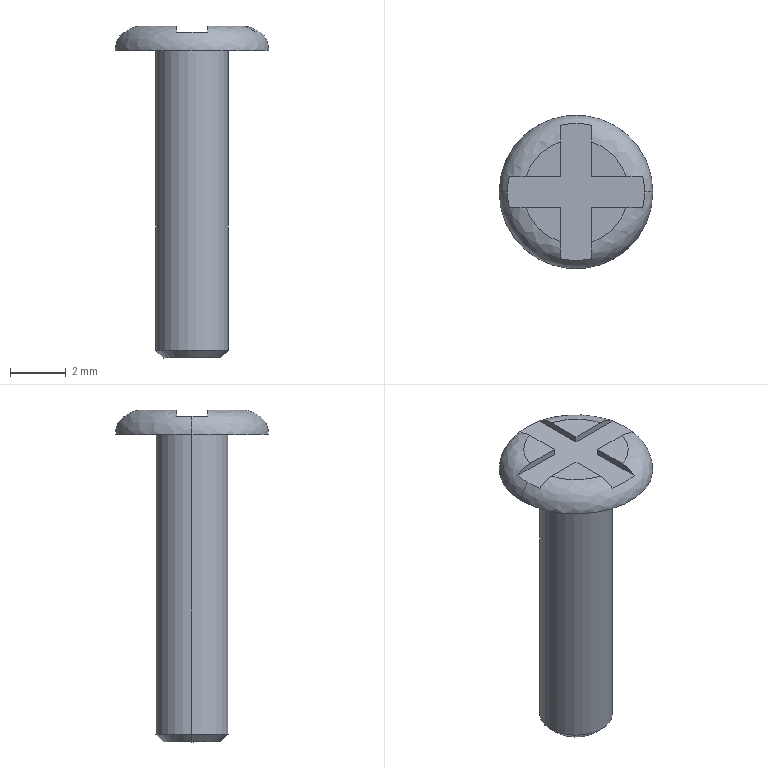Component | SolidWorks | NewCurveBenderHG20Slider-DoubleWheel-1_NewTypeCurveBenderHG20-DoubleWheel-1 | 1 solid | 21 faces | box 5.5 x 5.5 x 11.88 mm | volume 74 mm3 | plane 15 | spline 2 | cylinder 2 | cone 2 | commonest cylinder face diameters 2.6 x2
STEP:
#1=COLOUR_RGB('',0.7922,0.8196,0.9333);
#2=FILL_AREA_STYLE_COLOUR('',#1);
#3=FILL_AREA_STYLE('',(#2));
#4=SURFACE_STYLE_FILL_AREA(#3);
#5=SURFACE_SIDE_STYLE('',(#4));
#6=SURFACE_STYLE_USAGE(.BOTH.,#5);
#7=PRESENTATION_STYLE_ASSIGNMENT((#6));
#8=CARTESIAN_POINT('',(2.62,1.938,5.006));
#9=VERTEX_POINT('',#8);
#10=CARTESIAN_POINT('',(2.404,1.938,5.006));
#11=VERTEX_POINT('',#10);
#12=CARTESIAN_POINT('',(2.512,1.938,5.006));
#13=DIRECTION('',(-0.,0.,1.));
#14=DIRECTION('',(1.,0.,0.));
#15=AXIS2_PLACEMENT_3D('',#12,#13,#14);
#16=CIRCLE('',#15,0.1083);
#17=EDGE_CURVE('',#9,#11,#16,.T.);
#18=ORIENTED_EDGE('',*,*,#17,.T.);
#19=CARTESIAN_POINT('',(2.415,1.938,5.031));
#20=VERTEX_POINT('',#19);
#21=CARTESIAN_POINT('',(2.438,1.938,5.006));
#22=DIRECTION('',(-0.,1.,-0.));
#23=DIRECTION('',(-1.,0.,0.));
#24=AXIS2_PLACEMENT_3D('',#21,#22,#23);
#25=CIRCLE('',#24,0.03465);
#26=EDGE_CURVE('',#11,#20,#25,.T.);
#27=ORIENTED_EDGE('',*,*,#26,.T.);
#28=CARTESIAN_POINT('',(2.418,1.959,5.031));
#29=VERTEX_POINT('',#28);
#30=CARTESIAN_POINT('',(2.512,1.938,5.031));
#31=DIRECTION('',(0.,0.,-1.));
#32=DIRECTION('',(1.,0.,0.));
#33=AXIS2_PLACEMENT_3D('',#30,#31,#32);
#34=CIRCLE('',#33,0.09654);
#35=EDGE_CURVE('',#20,#29,#34,.T.);
#36=ORIENTED_EDGE('',*,*,#35,.T.);
#37=CARTESIAN_POINT('',(2.442,1.959,5.04));
#38=VERTEX_POINT('',#37);
#39=CARTESIAN_POINT('',(2.442,1.959,5.04));
#40=CARTESIAN_POINT('',(2.433,1.959,5.04));
#41=CARTESIAN_POINT('',(2.424,1.959,5.037));
#42=CARTESIAN_POINT('',(2.418,1.959,5.031));
#43=B_SPLINE_CURVE_WITH_KNOTS('',3,(#39,#40,#41,#42),.UNSPECIFIED.,.F.,.F.,(4,4),(0.,0.0006526),.UNSPECIFIED.);
#44=EDGE_CURVE('',#38,#29,#43,.T.);
#45=ORIENTED_EDGE('',*,*,#44,.F.);
#46=CARTESIAN_POINT('',(2.49,2.008,5.04));
#47=VERTEX_POINT('',#46);
#48=CARTESIAN_POINT('',(2.442,1.959,5.04));
#49=CARTESIAN_POINT('',(2.449,1.983,5.04));
#50=CARTESIAN_POINT('',(2.467,2.001,5.04));
#51=CARTESIAN_POINT('',(2.49,2.008,5.04));
#52=(BOUNDED_CURVE()B_SPLINE_CURVE(3,(#48,#49,#50,#51),.UNSPECIFIED.,.F.,.F.)B_SPLINE_CURVE_WITH_KNOTS((4,4),(0.,1.),.UNSPECIFIED.)CURVE()GEOMETRIC_REPRESENTATION_ITEM()RATIONAL_B_SPLINE_CURVE((1.,0.9225,0.9225,1.))REPRESENTATION_ITEM(''));
#53=EDGE_CURVE('',#38,#47,#52,.T.);
#54=ORIENTED_EDGE('',*,*,#53,.T.);
#55=CARTESIAN_POINT('',(2.49,2.032,5.031));
#56=VERTEX_POINT('',#55);
#57=CARTESIAN_POINT('',(2.49,2.032,5.031));
#58=CARTESIAN_POINT('',(2.49,2.025,5.037));
#59=CARTESIAN_POINT('',(2.49,2.017,5.04));
#60=CARTESIAN_POINT('',(2.49,2.008,5.04));
#61=B_SPLINE_CURVE_WITH_KNOTS('',3,(#57,#58,#59,#60),.UNSPECIFIED.,.F.,.F.,(4,4),(0.,0.0006513),.UNSPECIFIED.);
#62=EDGE_CURVE('',#56,#47,#61,.T.);
#63=ORIENTED_EDGE('',*,*,#62,.F.);
#64=CARTESIAN_POINT('',(2.534,2.032,5.031));
#65=VERTEX_POINT('',#64);
#66=CARTESIAN_POINT('',(2.512,1.938,5.031));
#67=DIRECTION('',(0.,0.,-1.));
#68=DIRECTION('',(1.,0.,0.));
#69=AXIS2_PLACEMENT_3D('',#66,#67,#68);
#70=CIRCLE('',#69,0.09654);
#71=EDGE_CURVE('',#56,#65,#70,.T.);
#72=ORIENTED_EDGE('',*,*,#71,.T.);
#73=CARTESIAN_POINT('',(2.534,2.008,5.04));
#74=VERTEX_POINT('',#73);
#75=CARTESIAN_POINT('',(2.534,2.008,5.04));
#76=CARTESIAN_POINT('',(2.534,2.017,5.04));
#77=CARTESIAN_POINT('',(2.534,2.025,5.037));
#78=CARTESIAN_POINT('',(2.534,2.032,5.031));
#79=B_SPLINE_CURVE_WITH_KNOTS('',3,(#75,#76,#77,#78),.UNSPECIFIED.,.F.,.F.,(4,4),(0.,0.0006526),.UNSPECIFIED.);
#80=EDGE_CURVE('',#74,#65,#79,.T.);
#81=ORIENTED_EDGE('',*,*,#80,.F.);
#82=CARTESIAN_POINT('',(2.582,1.959,5.04));
#83=VERTEX_POINT('',#82);
#84=CARTESIAN_POINT('',(2.534,2.008,5.04));
#85=CARTESIAN_POINT('',(2.557,2.001,5.04));
#86=CARTESIAN_POINT('',(2.575,1.983,5.04));
#87=CARTESIAN_POINT('',(2.582,1.959,5.04));
#88=(BOUNDED_CURVE()B_SPLINE_CURVE(3,(#84,#85,#86,#87),.UNSPECIFIED.,.F.,.F.)B_SPLINE_CURVE_WITH_KNOTS((4,4),(0.,1.),.UNSPECIFIED.)CURVE()GEOMETRIC_REPRESENTATION_ITEM()RATIONAL_B_SPLINE_CURVE((1.,0.9225,0.9225,1.))REPRESENTATION_ITEM(''));
#89=EDGE_CURVE('',#74,#83,#88,.T.);
#90=ORIENTED_EDGE('',*,*,#89,.T.);
#91=CARTESIAN_POINT('',(2.606,1.959,5.031));
#92=VERTEX_POINT('',#91);
#93=CARTESIAN_POINT('',(2.606,1.959,5.031));
#94=CARTESIAN_POINT('',(2.599,1.959,5.037));
#95=CARTESIAN_POINT('',(2.591,1.959,5.04));
#96=CARTESIAN_POINT('',(2.582,1.959,5.04));
#97=B_SPLINE_CURVE_WITH_KNOTS('',3,(#93,#94,#95,#96),.UNSPECIFIED.,.F.,.F.,(4,4),(0.,0.0006513),.UNSPECIFIED.);
#98=EDGE_CURVE('',#92,#83,#97,.T.);
#99=ORIENTED_EDGE('',*,*,#98,.F.);
#100=CARTESIAN_POINT('',(2.609,1.938,5.031));
#101=VERTEX_POINT('',#100);
#102=CARTESIAN_POINT('',(2.512,1.938,5.031));
#103=DIRECTION('',(0.,0.,-1.));
#104=DIRECTION('',(1.,0.,0.));
#105=AXIS2_PLACEMENT_3D('',#102,#103,#104);
#106=CIRCLE('',#105,0.09654);
#107=EDGE_CURVE('',#92,#101,#106,.T.);
#108=ORIENTED_EDGE('',*,*,#107,.T.);
#109=CARTESIAN_POINT('',(2.586,1.938,5.006));
#110=DIRECTION('',(0.,-1.,0.));
#111=DIRECTION('',(1.,0.,0.));
#112=AXIS2_PLACEMENT_3D('',#109,#110,#111);
#113=CIRCLE('',#112,0.03465);
#114=EDGE_CURVE('',#9,#101,#113,.T.);
#115=ORIENTED_EDGE('',*,*,#114,.F.);
#116=EDGE_LOOP('',(#18,#27,#36,#45,#54,#63,#72,#81,#90,#99,#108,#115));
#117=FACE_OUTER_BOUND('',#116,.T.);
#118=CARTESIAN_POINT('',(2.404,1.938,5.006));
#119=CARTESIAN_POINT('',(2.404,2.154,5.006));
#120=CARTESIAN_POINT('',(2.62,2.154,5.006));
#121=CARTESIAN_POINT('',(2.62,1.938,5.006));
#122=CARTESIAN_POINT('',(2.404,1.938,5.026));
#123=CARTESIAN_POINT('',(2.404,2.154,5.026));
#124=CARTESIAN_POINT('',(2.62,2.154,5.026));
#125=CARTESIAN_POINT('',(2.62,1.938,5.026));
#126=CARTESIAN_POINT('',(2.418,1.938,5.04));
#127=CARTESIAN_POINT('',(2.418,2.125,5.04));
#128=CARTESIAN_POINT('',(2.606,2.125,5.04));
#129=CARTESIAN_POINT('',(2.606,1.938,5.04));
#130=CARTESIAN_POINT('',(2.438,1.938,5.04));
#131=CARTESIAN_POINT('',(2.438,2.085,5.04));
#132=CARTESIAN_POINT('',(2.586,2.085,5.04));
#133=CARTESIAN_POINT('',(2.586,1.938,5.04));
#134=(BOUNDED_SURFACE()B_SPLINE_SURFACE(3,3,((#118,#119,#120,#121),(#122,#123,#124,#125),(#126,#127,#128,#129),(#130,#131,#132,#133)),.UNSPECIFIED.,.F.,.F.,.F.)B_SPLINE_SURFACE_WITH_KNOTS((4,4),(4,4),(0.,1.),(0.,1.),.UNSPECIFIED.)GEOMETRIC_REPRESENTATION_ITEM()RATIONAL_B_SPLINE_SURFACE(((1.,0.3333,0.3333,1.),(0.8047,0.2682,0.2682,0.8047),(0.8047,0.2682,0.2682,0.8047),(1.,0.3333,0.3333,1.)))REPRESENTATION_ITEM('')SURFACE());
#135=ADVANCED_FACE('',(#117),#134,.T.);
#136=CARTESIAN_POINT('',(2.461,1.938,4.583));
#137=VERTEX_POINT('',#136);
#138=CARTESIAN_POINT('',(2.563,1.938,4.583));
#139=VERTEX_POINT('',#138);
#140=CARTESIAN_POINT('',(2.512,1.938,4.583));
#141=DIRECTION('',(-0.,0.,1.));
#142=DIRECTION('',(-1.,0.,-0.));
#143=AXIS2_PLACEMENT_3D('',#140,#141,#142);
#144=CIRCLE('',#143,0.05118);
#145=EDGE_CURVE('',#137,#139,#144,.T.);
#146=ORIENTED_EDGE('',*,*,#145,.T.);
#147=CARTESIAN_POINT('',(2.563,1.938,5.006));
#148=VERTEX_POINT('',#147);
#149=CARTESIAN_POINT('',(2.563,1.938,4.572));
#150=DIRECTION('',(-0.,0.,1.));
#151=VECTOR('',#150,39.37);
#152=LINE('',#149,#151);
#153=EDGE_CURVE('',#139,#148,#152,.T.);
#154=ORIENTED_EDGE('',*,*,#153,.T.);
#155=CARTESIAN_POINT('',(2.461,1.938,5.006));
#156=VERTEX_POINT('',#155);
#157=CARTESIAN_POINT('',(2.512,1.938,5.006));
#158=DIRECTION('',(0.,0.,-1.));
#159=DIRECTION('',(-1.,0.,0.));
#160=AXIS2_PLACEMENT_3D('',#157,#158,#159);
#161=CIRCLE('',#160,0.05118);
#162=EDGE_CURVE('',#148,#156,#161,.T.);
#163=ORIENTED_EDGE('',*,*,#162,.T.);
#164=CARTESIAN_POINT('',(2.461,1.938,4.572));
#165=DIRECTION('',(-0.,0.,1.));
#166=VECTOR('',#165,39.37);
#167=LINE('',#164,#166);
#168=EDGE_CURVE('',#137,#156,#167,.T.);
#169=ORIENTED_EDGE('',*,*,#168,.F.);
#170=EDGE_LOOP('',(#146,#154,#163,#169));
#171=FACE_OUTER_BOUND('',#170,.T.);
#172=CARTESIAN_POINT('',(2.512,1.938,4.572));
#173=DIRECTION('',(-0.,0.,1.));
#174=DIRECTION('',(-1.,0.,-0.));
#175=AXIS2_PLACEMENT_3D('',#172,#173,#174);
#176=CYLINDRICAL_SURFACE('',#175,0.05118);
#177=ADVANCED_FACE('',(#171),#176,.T.);
#178=CARTESIAN_POINT('',(2.472,1.938,4.572));
#179=VERTEX_POINT('',#178);
#180=CARTESIAN_POINT('',(2.552,1.938,4.572));
#181=VERTEX_POINT('',#180);
#182=CARTESIAN_POINT('',(2.512,1.938,4.572));
#183=DIRECTION('',(-0.,0.,1.));
#184=DIRECTION('',(-1.,0.,-0.));
#185=AXIS2_PLACEMENT_3D('',#182,#183,#184);
#186=CIRCLE('',#185,0.04031);
#187=EDGE_CURVE('',#179,#181,#186,.T.);
#188=ORIENTED_EDGE('',*,*,#187,.T.);
#189=CARTESIAN_POINT('',(2.563,1.938,4.583));
#190=DIRECTION('',(0.7071,-0.,0.7071));
#191=VECTOR('',#190,39.37);
#192=LINE('',#189,#191);
#193=EDGE_CURVE('',#181,#139,#192,.T.);
#194=ORIENTED_EDGE('',*,*,#193,.T.);
#195=ORIENTED_EDGE('',*,*,#145,.F.);
#196=CARTESIAN_POINT('',(2.461,1.938,4.583));
#197=DIRECTION('',(-0.7071,0.,0.7071));
#198=VECTOR('',#197,39.37);
#199=LINE('',#196,#198);
#200=EDGE_CURVE('',#179,#137,#199,.T.);
#201=ORIENTED_EDGE('',*,*,#200,.F.);
#202=EDGE_LOOP('',(#188,#194,#195,#201));
#203=FACE_OUTER_BOUND('',#202,.T.);
#204=CARTESIAN_POINT('',(2.512,1.938,4.583));
#205=DIRECTION('',(-0.,0.,1.));
#206=DIRECTION('',(-1.,0.,-0.));
#207=AXIS2_PLACEMENT_3D('',#204,#205,#206);
#208=CONICAL_SURFACE('',#207,0.05118,0.7854);
#209=ADVANCED_FACE('',(#203),#208,.T.);
#210=ORIENTED_EDGE('',*,*,#153,.F.);
#211=CARTESIAN_POINT('',(2.512,1.938,4.583));
#212=DIRECTION('',(-0.,0.,1.));
#213=DIRECTION('',(-1.,0.,-0.));
#214=AXIS2_PLACEMENT_3D('',#211,#212,#213);
#215=CIRCLE('',#214,0.05118);
#216=EDGE_CURVE('',#139,#137,#215,.T.);
#217=ORIENTED_EDGE('',*,*,#216,.T.);
#218=ORIENTED_EDGE('',*,*,#168,.T.);
#219=CARTESIAN_POINT('',(2.512,1.938,5.006));
#220=DIRECTION('',(0.,0.,-1.));
#221=DIRECTION('',(-1.,0.,0.));
#222=AXIS2_PLACEMENT_3D('',#219,#220,#221);
#223=CIRCLE('',#222,0.05118);
#224=EDGE_CURVE('',#156,#148,#223,.T.);
#225=ORIENTED_EDGE('',*,*,#224,.T.);
#226=EDGE_LOOP('',(#210,#217,#218,#225));
#227=FACE_OUTER_BOUND('',#226,.T.);
#228=CARTESIAN_POINT('',(2.512,1.938,4.572));
#229=DIRECTION('',(-0.,0.,1.));
#230=DIRECTION('',(-1.,0.,-0.));
#231=AXIS2_PLACEMENT_3D('',#228,#229,#230);
#232=CYLINDRICAL_SURFACE('',#231,0.05118);
#233=ADVANCED_FACE('',(#227),#232,.T.);
#234=ORIENTED_EDGE('',*,*,#17,.F.);
#235=CARTESIAN_POINT('',(2.512,1.938,5.006));
#236=DIRECTION('',(-0.,0.,1.));
#237=DIRECTION('',(1.,0.,0.));
#238=AXIS2_PLACEMENT_3D('',#235,#236,#237);
#239=CIRCLE('',#238,0.1083);
#240=EDGE_CURVE('',#11,#9,#239,.T.);
#241=ORIENTED_EDGE('',*,*,#240,.F.);
#242=EDGE_LOOP('',(#234,#241));
#243=FACE_OUTER_BOUND('',#242,.T.);
#244=ORIENTED_EDGE('',*,*,#224,.F.);
#245=ORIENTED_EDGE('',*,*,#162,.F.);
#246=EDGE_LOOP('',(#244,#245));
#247=FACE_BOUND('',#246,.T.);
#248=CARTESIAN_POINT('',(2.512,1.829,5.006));
#249=DIRECTION('',(-0.,0.,1.));
#250=DIRECTION('',(-1.,0.,-0.));
#251=AXIS2_PLACEMENT_3D('',#248,#249,#250);
#252=PLANE('',#251);
#253=ADVANCED_FACE('',(#243,#247),#252,.F.);
#254=ORIENTED_EDGE('',*,*,#193,.F.);
#255=CARTESIAN_POINT('',(2.512,1.938,4.572));
#256=DIRECTION('',(-0.,0.,1.));
#257=DIRECTION('',(-1.,0.,-0.));
#258=AXIS2_PLACEMENT_3D('',#255,#256,#257);
#259=CIRCLE('',#258,0.04031);
#260=EDGE_CURVE('',#181,#179,#259,.T.);
#261=ORIENTED_EDGE('',*,*,#260,.T.);
#262=ORIENTED_EDGE('',*,*,#200,.T.);
#263=ORIENTED_EDGE('',*,*,#216,.F.);
#264=EDGE_LOOP('',(#254,#261,#262,#263));
#265=FACE_OUTER_BOUND('',#264,.T.);
#266=CARTESIAN_POINT('',(2.512,1.938,4.583));
#267=DIRECTION('',(-0.,0.,1.));
#268=DIRECTION('',(-1.,0.,-0.));
#269=AXIS2_PLACEMENT_3D('',#266,#267,#268);
#270=CONICAL_SURFACE('',#269,0.05118,0.7854);
#271=ADVANCED_FACE('',(#265),#270,.T.);
#272=ORIENTED_EDGE('',*,*,#26,.F.);
#273=ORIENTED_EDGE('',*,*,#240,.T.);
#274=ORIENTED_EDGE('',*,*,#114,.T.);
#275=CARTESIAN_POINT('',(2.606,1.916,5.031));
#276=VERTEX_POINT('',#275);
#277=CARTESIAN_POINT('',(2.512,1.938,5.031));
#278=DIRECTION('',(0.,0.,-1.));
#279=DIRECTION('',(1.,0.,0.));
#280=AXIS2_PLACEMENT_3D('',#277,#278,#279);
#281=CIRCLE('',#280,0.09654);
#282=EDGE_CURVE('',#101,#276,#281,.T.);
#283=ORIENTED_EDGE('',*,*,#282,.T.);
#284=CARTESIAN_POINT('',(2.582,1.916,5.04));
#285=VERTEX_POINT('',#284);
#286=CARTESIAN_POINT('',(2.582,1.916,5.04));
#287=CARTESIAN_POINT('',(2.591,1.916,5.04));
#288=CARTESIAN_POINT('',(2.599,1.916,5.037));
#289=CARTESIAN_POINT('',(2.606,1.916,5.031));
#290=B_SPLINE_CURVE_WITH_KNOTS('',3,(#286,#287,#288,#289),.UNSPECIFIED.,.F.,.F.,(4,4),(0.,0.0006526),.UNSPECIFIED.);
#291=EDGE_CURVE('',#285,#276,#290,.T.);
#292=ORIENTED_EDGE('',*,*,#291,.F.);
#293=CARTESIAN_POINT('',(2.534,1.867,5.04));
#294=VERTEX_POINT('',#293);
#295=CARTESIAN_POINT('',(2.582,1.916,5.04));
#296=CARTESIAN_POINT('',(2.575,1.892,5.04));
#297=CARTESIAN_POINT('',(2.557,1.875,5.04));
#298=CARTESIAN_POINT('',(2.534,1.867,5.04));
#299=(BOUNDED_CURVE()B_SPLINE_CURVE(3,(#295,#296,#297,#298),.UNSPECIFIED.,.F.,.F.)B_SPLINE_CURVE_WITH_KNOTS((4,4),(0.,1.),.UNSPECIFIED.)CURVE()GEOMETRIC_REPRESENTATION_ITEM()RATIONAL_B_SPLINE_CURVE((1.,0.9225,0.9225,1.))REPRESENTATION_ITEM(''));
#300=EDGE_CURVE('',#285,#294,#299,.T.);
#301=ORIENTED_EDGE('',*,*,#300,.T.);
#302=CARTESIAN_POINT('',(2.534,1.844,5.031));
#303=VERTEX_POINT('',#302);
#304=CARTESIAN_POINT('',(2.534,1.844,5.031));
#305=CARTESIAN_POINT('',(2.534,1.85,5.037));
#306=CARTESIAN_POINT('',(2.534,1.859,5.04));
#307=CARTESIAN_POINT('',(2.534,1.867,5.04));
#308=B_SPLINE_CURVE_WITH_KNOTS('',3,(#304,#305,#306,#307),.UNSPECIFIED.,.F.,.F.,(4,4),(0.,0.0006513),.UNSPECIFIED.);
#309=EDGE_CURVE('',#303,#294,#308,.T.);
#310=ORIENTED_EDGE('',*,*,#309,.F.);
#311=CARTESIAN_POINT('',(2.49,1.844,5.031));
#312=VERTEX_POINT('',#311);
#313=CARTESIAN_POINT('',(2.512,1.938,5.031));
#314=DIRECTION('',(0.,0.,-1.));
#315=DIRECTION('',(1.,0.,0.));
#316=AXIS2_PLACEMENT_3D('',#313,#314,#315);
#317=CIRCLE('',#316,0.09654);
#318=EDGE_CURVE('',#303,#312,#317,.T.);
#319=ORIENTED_EDGE('',*,*,#318,.T.);
#320=CARTESIAN_POINT('',(2.49,1.867,5.04));
#321=VERTEX_POINT('',#320);
#322=CARTESIAN_POINT('',(2.49,1.844,5.031));
#323=CARTESIAN_POINT('',(2.49,1.85,5.037));
#324=CARTESIAN_POINT('',(2.49,1.859,5.04));
#325=CARTESIAN_POINT('',(2.49,1.867,5.04));
#326=B_SPLINE_CURVE_WITH_KNOTS('',3,(#322,#323,#324,#325),.UNSPECIFIED.,.F.,.F.,(4,4),(0.,0.0006513),.UNSPECIFIED.);
#327=EDGE_CURVE('',#312,#321,#326,.T.);
#328=ORIENTED_EDGE('',*,*,#327,.T.);
#329=CARTESIAN_POINT('',(2.442,1.916,5.04));
#330=VERTEX_POINT('',#329);
#331=CARTESIAN_POINT('',(2.49,1.867,5.04));
#332=CARTESIAN_POINT('',(2.467,1.875,5.04));
#333=CARTESIAN_POINT('',(2.449,1.892,5.04));
#334=CARTESIAN_POINT('',(2.442,1.916,5.04));
#335=(BOUNDED_CURVE()B_SPLINE_CURVE(3,(#331,#332,#333,#334),.UNSPECIFIED.,.F.,.F.)B_SPLINE_CURVE_WITH_KNOTS((4,4),(0.,1.),.UNSPECIFIED.)CURVE()GEOMETRIC_REPRESENTATION_ITEM()RATIONAL_B_SPLINE_CURVE((1.,0.9225,0.9225,1.))REPRESENTATION_ITEM(''));
#336=EDGE_CURVE('',#321,#330,#335,.T.);
#337=ORIENTED_EDGE('',*,*,#336,.T.);
#338=CARTESIAN_POINT('',(2.418,1.916,5.031));
#339=VERTEX_POINT('',#338);
#340=CARTESIAN_POINT('',(2.418,1.916,5.031));
#341=CARTESIAN_POINT('',(2.424,1.916,5.037));
#342=CARTESIAN_POINT('',(2.433,1.916,5.04));
#343=CARTESIAN_POINT('',(2.442,1.916,5.04));
#344=B_SPLINE_CURVE_WITH_KNOTS('',3,(#340,#341,#342,#343),.UNSPECIFIED.,.F.,.F.,(4,4),(0.,0.0006513),.UNSPECIFIED.);
#345=EDGE_CURVE('',#339,#330,#344,.T.);
#346=ORIENTED_EDGE('',*,*,#345,.F.);
#347=CARTESIAN_POINT('',(2.512,1.938,5.031));
#348=DIRECTION('',(0.,0.,-1.));
#349=DIRECTION('',(1.,0.,0.));
#350=AXIS2_PLACEMENT_3D('',#347,#348,#349);
#351=CIRCLE('',#350,0.09654);
#352=EDGE_CURVE('',#339,#20,#351,.T.);
#353=ORIENTED_EDGE('',*,*,#352,.T.);
#354=EDGE_LOOP('',(#272,#273,#274,#283,#292,#301,#310,#319,#328,#337,#346,#353));
#355=FACE_OUTER_BOUND('',#354,.T.);
#356=CARTESIAN_POINT('',(2.62,1.938,5.006));
#357=CARTESIAN_POINT('',(2.62,1.721,5.006));
#358=CARTESIAN_POINT('',(2.404,1.721,5.006));
#359=CARTESIAN_POINT('',(2.404,1.938,5.006));
#360=CARTESIAN_POINT('',(2.62,1.938,5.026));
#361=CARTESIAN_POINT('',(2.62,1.721,5.026));
#362=CARTESIAN_POINT('',(2.404,1.721,5.026));
#363=CARTESIAN_POINT('',(2.404,1.938,5.026));
#364=CARTESIAN_POINT('',(2.606,1.938,5.04));
#365=CARTESIAN_POINT('',(2.606,1.75,5.04));
#366=CARTESIAN_POINT('',(2.418,1.75,5.04));
#367=CARTESIAN_POINT('',(2.418,1.938,5.04));
#368=CARTESIAN_POINT('',(2.586,1.938,5.04));
#369=CARTESIAN_POINT('',(2.586,1.79,5.04));
#370=CARTESIAN_POINT('',(2.438,1.79,5.04));
#371=CARTESIAN_POINT('',(2.438,1.938,5.04));
#372=(BOUNDED_SURFACE()B_SPLINE_SURFACE(3,3,((#356,#357,#358,#359),(#360,#361,#362,#363),(#364,#365,#366,#367),(#368,#369,#370,#371)),.UNSPECIFIED.,.F.,.F.,.F.)B_SPLINE_SURFACE_WITH_KNOTS((4,4),(4,4),(0.,1.),(0.,1.),.UNSPECIFIED.)GEOMETRIC_REPRESENTATION_ITEM()RATIONAL_B_SPLINE_SURFACE(((1.,0.3333,0.3333,1.),(0.8047,0.2682,0.2682,0.8047),(0.8047,0.2682,0.2682,0.8047),(1.,0.3333,0.3333,1.)))REPRESENTATION_ITEM('')SURFACE());
#373=ADVANCED_FACE('',(#355),#372,.T.);
#374=ORIENTED_EDGE('',*,*,#187,.F.);
#375=ORIENTED_EDGE('',*,*,#260,.F.);
#376=EDGE_LOOP('',(#374,#375));
#377=FACE_OUTER_BOUND('',#376,.T.);
#378=CARTESIAN_POINT('',(2.512,1.897,4.572));
#379=DIRECTION('',(-0.,0.,1.));
#380=DIRECTION('',(-1.,0.,-0.));
#381=AXIS2_PLACEMENT_3D('',#378,#379,#380);
#382=PLANE('',#381);
#383=ADVANCED_FACE('',(#377),#382,.F.);
#384=CARTESIAN_POINT('',(2.534,1.916,5.04));
#385=VERTEX_POINT('',#384);
#386=CARTESIAN_POINT('',(2.534,1.916,5.04));
#387=DIRECTION('',(0.,1.,0.));
#388=VECTOR('',#387,39.37);
#389=LINE('',#386,#388);
#390=EDGE_CURVE('',#294,#385,#389,.T.);
#391=ORIENTED_EDGE('',*,*,#390,.F.);
#392=ORIENTED_EDGE('',*,*,#300,.F.);
#393=CARTESIAN_POINT('',(2.618,1.916,5.04));
#394=DIRECTION('',(1.,0.,0.));
#395=VECTOR('',#394,39.37);
#396=LINE('',#393,#395);
#397=EDGE_CURVE('',#385,#285,#396,.T.);
#398=ORIENTED_EDGE('',*,*,#397,.F.);
#399=EDGE_LOOP('',(#391,#392,#398));
#400=FACE_OUTER_BOUND('',#399,.T.);
#401=CARTESIAN_POINT('',(2.512,1.938,5.04));
#402=DIRECTION('',(0.,0.,-1.));
#403=DIRECTION('',(1.,0.,0.));
#404=AXIS2_PLACEMENT_3D('',#401,#402,#403);
#405=PLANE('',#404);
#406=ADVANCED_FACE('',(#400),#405,.F.);
#407=CARTESIAN_POINT('',(2.534,1.959,5.04));
#408=VERTEX_POINT('',#407);
#409=CARTESIAN_POINT('',(2.534,1.959,5.04));
#410=DIRECTION('',(-1.,-0.,-0.));
#411=VECTOR('',#410,39.37);
#412=LINE('',#409,#411);
#413=EDGE_CURVE('',#83,#408,#412,.T.);
#414=ORIENTED_EDGE('',*,*,#413,.F.);
#415=ORIENTED_EDGE('',*,*,#89,.F.);
#416=CARTESIAN_POINT('',(2.534,2.044,5.04));
#417=DIRECTION('',(0.,1.,0.));
#418=VECTOR('',#417,39.37);
#419=LINE('',#416,#418);
#420=EDGE_CURVE('',#408,#74,#419,.T.);
#421=ORIENTED_EDGE('',*,*,#420,.F.);
#422=EDGE_LOOP('',(#414,#415,#421));
#423=FACE_OUTER_BOUND('',#422,.T.);
#424=CARTESIAN_POINT('',(2.512,1.938,5.04));
#425=DIRECTION('',(0.,0.,-1.));
#426=DIRECTION('',(1.,0.,0.));
#427=AXIS2_PLACEMENT_3D('',#424,#425,#426);
#428=PLANE('',#427);
#429=ADVANCED_FACE('',(#423),#428,.F.);
#430=CARTESIAN_POINT('',(2.49,1.959,5.04));
#431=VERTEX_POINT('',#430);
#432=CARTESIAN_POINT('',(2.49,1.959,5.04));
#433=DIRECTION('',(0.,-1.,0.));
#434=VECTOR('',#433,39.37);
#435=LINE('',#432,#434);
#436=EDGE_CURVE('',#47,#431,#435,.T.);
#437=ORIENTED_EDGE('',*,*,#436,.F.);
#438=ORIENTED_EDGE('',*,*,#53,.F.);
#439=CARTESIAN_POINT('',(2.406,1.959,5.04));
#440=DIRECTION('',(-1.,0.,-0.));
#441=VECTOR('',#440,39.37);
#442=LINE('',#439,#441);
#443=EDGE_CURVE('',#431,#38,#442,.T.);
#444=ORIENTED_EDGE('',*,*,#443,.F.);
#445=EDGE_LOOP('',(#437,#438,#444));
#446=FACE_OUTER_BOUND('',#445,.T.);
#447=CARTESIAN_POINT('',(2.512,1.938,5.04));
#448=DIRECTION('',(0.,0.,-1.));
#449=DIRECTION('',(1.,0.,0.));
#450=AXIS2_PLACEMENT_3D('',#447,#448,#449);
#451=PLANE('',#450);
#452=ADVANCED_FACE('',(#446),#451,.F.);
#453=ORIENTED_EDGE('',*,*,#336,.F.);
#454=CARTESIAN_POINT('',(2.49,1.916,5.04));
#455=VERTEX_POINT('',#454);
#456=CARTESIAN_POINT('',(2.49,1.938,5.04));
#457=DIRECTION('',(0.,-1.,0.));
#458=VECTOR('',#457,39.37);
#459=LINE('',#456,#458);
#460=EDGE_CURVE('',#455,#321,#459,.T.);
#461=ORIENTED_EDGE('',*,*,#460,.F.);
#462=CARTESIAN_POINT('',(2.49,1.916,5.04));
#463=DIRECTION('',(1.,0.,0.));
#464=VECTOR('',#463,39.37);
#465=LINE('',#462,#464);
#466=EDGE_CURVE('',#330,#455,#465,.T.);
#467=ORIENTED_EDGE('',*,*,#466,.F.);
#468=EDGE_LOOP('',(#453,#461,#467));
#469=FACE_OUTER_BOUND('',#468,.T.);
#470=CARTESIAN_POINT('',(2.512,1.938,5.04));
#471=DIRECTION('',(0.,0.,-1.));
#472=DIRECTION('',(1.,0.,0.));
#473=AXIS2_PLACEMENT_3D('',#470,#471,#472);
#474=PLANE('',#473);
#475=ADVANCED_FACE('',(#469),#474,.F.);
#476=ORIENTED_EDGE('',*,*,#460,.T.);
#477=ORIENTED_EDGE('',*,*,#327,.F.);
#478=CARTESIAN_POINT('',(2.49,1.916,5.031));
#479=VERTEX_POINT('',#478);
#480=CARTESIAN_POINT('',(2.49,1.832,5.031));
#481=DIRECTION('',(0.,1.,0.));
#482=VECTOR('',#481,39.37);
#483=LINE('',#480,#482);
#484=EDGE_CURVE('',#312,#479,#483,.T.);
#485=ORIENTED_EDGE('',*,*,#484,.T.);
#486=CARTESIAN_POINT('',(2.49,1.916,5.031));
#487=DIRECTION('',(0.,0.,-1.));
#488=VECTOR('',#487,39.37);
#489=LINE('',#486,#488);
#490=EDGE_CURVE('',#455,#479,#489,.T.);
#491=ORIENTED_EDGE('',*,*,#490,.F.);
#492=EDGE_LOOP('',(#476,#477,#485,#491));
#493=FACE_OUTER_BOUND('',#492,.T.);
#494=CARTESIAN_POINT('',(2.49,1.832,5.031));
#495=DIRECTION('',(1.,0.,0.));
#496=DIRECTION('',(-0.,0.,1.));
#497=AXIS2_PLACEMENT_3D('',#494,#495,#496);
#498=PLANE('',#497);
#499=ADVANCED_FACE('',(#493),#498,.T.);
#500=CARTESIAN_POINT('',(2.49,1.959,5.031));
#501=VERTEX_POINT('',#500);
#502=CARTESIAN_POINT('',(2.49,1.938,5.031));
#503=DIRECTION('',(0.,1.,0.));
#504=VECTOR('',#503,39.37);
#505=LINE('',#502,#504);
#506=EDGE_CURVE('',#501,#56,#505,.T.);
#507=ORIENTED_EDGE('',*,*,#506,.F.);
#508=CARTESIAN_POINT('',(2.512,1.959,5.031));
#509=DIRECTION('',(1.,0.,0.));
#510=VECTOR('',#509,39.37);
#511=LINE('',#508,#510);
#512=EDGE_CURVE('',#29,#501,#511,.T.);
#513=ORIENTED_EDGE('',*,*,#512,.F.);
#514=ORIENTED_EDGE('',*,*,#35,.F.);
#515=ORIENTED_EDGE('',*,*,#352,.F.);
#516=CARTESIAN_POINT('',(2.512,1.916,5.031));
#517=DIRECTION('',(-1.,0.,-0.));
#518=VECTOR('',#517,39.37);
#519=LINE('',#516,#518);
#520=EDGE_CURVE('',#479,#339,#519,.T.);
#521=ORIENTED_EDGE('',*,*,#520,.F.);
#522=ORIENTED_EDGE('',*,*,#484,.F.);
#523=ORIENTED_EDGE('',*,*,#318,.F.);
#524=CARTESIAN_POINT('',(2.534,1.916,5.031));
#525=VERTEX_POINT('',#524);
#526=CARTESIAN_POINT('',(2.534,1.938,5.031));
#527=DIRECTION('',(0.,-1.,0.));
#528=VECTOR('',#527,39.37);
#529=LINE('',#526,#528);
#530=EDGE_CURVE('',#525,#303,#529,.T.);
#531=ORIENTED_EDGE('',*,*,#530,.F.);
#532=CARTESIAN_POINT('',(2.512,1.916,5.031));
#533=DIRECTION('',(-1.,0.,-0.));
#534=VECTOR('',#533,39.37);
#535=LINE('',#532,#534);
#536=EDGE_CURVE('',#276,#525,#535,.T.);
#537=ORIENTED_EDGE('',*,*,#536,.F.);
#538=ORIENTED_EDGE('',*,*,#282,.F.);
#539=ORIENTED_EDGE('',*,*,#107,.F.);
#540=CARTESIAN_POINT('',(2.534,1.959,5.031));
#541=VERTEX_POINT('',#540);
#542=CARTESIAN_POINT('',(2.512,1.959,5.031));
#543=DIRECTION('',(1.,0.,0.));
#544=VECTOR('',#543,39.37);
#545=LINE('',#542,#544);
#546=EDGE_CURVE('',#541,#92,#545,.T.);
#547=ORIENTED_EDGE('',*,*,#546,.F.);
#548=CARTESIAN_POINT('',(2.534,1.938,5.031));
#549=DIRECTION('',(0.,-1.,0.));
#550=VECTOR('',#549,39.37);
#551=LINE('',#548,#550);
#552=EDGE_CURVE('',#65,#541,#551,.T.);
#553=ORIENTED_EDGE('',*,*,#552,.F.);
#554=ORIENTED_EDGE('',*,*,#71,.F.);
#555=EDGE_LOOP('',(#507,#513,#514,#515,#521,#522,#523,#531,#537,#538,#539,#547,#553,#554));
#556=FACE_OUTER_BOUND('',#555,.T.);
#557=CARTESIAN_POINT('',(2.512,1.938,5.031));
#558=DIRECTION('',(0.,0.,-1.));
#559=DIRECTION('',(1.,0.,0.));
#560=AXIS2_PLACEMENT_3D('',#557,#558,#559);
#561=PLANE('',#560);
#562=ADVANCED_FACE('',(#556),#561,.F.);
#563=ORIENTED_EDGE('',*,*,#506,.T.);
#564=ORIENTED_EDGE('',*,*,#62,.T.);
#565=ORIENTED_EDGE('',*,*,#436,.T.);
#566=CARTESIAN_POINT('',(2.49,1.959,5.031));
#567=DIRECTION('',(0.,0.,-1.));
#568=VECTOR('',#567,39.37);
#569=LINE('',#566,#568);
#570=EDGE_CURVE('',#431,#501,#569,.T.);
#571=ORIENTED_EDGE('',*,*,#570,.T.);
#572=EDGE_LOOP('',(#563,#564,#565,#571));
#573=FACE_OUTER_BOUND('',#572,.T.);
#574=CARTESIAN_POINT('',(2.49,1.959,5.031));
#575=DIRECTION('',(1.,0.,0.));
#576=DIRECTION('',(0.,-1.,0.));
#577=AXIS2_PLACEMENT_3D('',#574,#575,#576);
#578=PLANE('',#577);
#579=ADVANCED_FACE('',(#573),#578,.T.);
#580=ORIENTED_EDGE('',*,*,#443,.T.);
#581=ORIENTED_EDGE('',*,*,#44,.T.);
#582=ORIENTED_EDGE('',*,*,#512,.T.);
#583=ORIENTED_EDGE('',*,*,#570,.F.);
#584=EDGE_LOOP('',(#580,#581,#582,#583));
#585=FACE_OUTER_BOUND('',#584,.T.);
#586=CARTESIAN_POINT('',(2.406,1.959,5.031));
#587=DIRECTION('',(0.,-1.,0.));
#588=DIRECTION('',(-1.,0.,-0.));
#589=AXIS2_PLACEMENT_3D('',#586,#587,#588);
#590=PLANE('',#589);
#591=ADVANCED_FACE('',(#585),#590,.T.);
#592=ORIENTED_EDGE('',*,*,#520,.T.);
#593=ORIENTED_EDGE('',*,*,#345,.T.);
#594=ORIENTED_EDGE('',*,*,#466,.T.);
#595=ORIENTED_EDGE('',*,*,#490,.T.);
#596=EDGE_LOOP('',(#592,#593,#594,#595));
#597=FACE_OUTER_BOUND('',#596,.T.);
#598=CARTESIAN_POINT('',(2.49,1.916,5.031));
#599=DIRECTION('',(-0.,1.,-0.));
#600=DIRECTION('',(1.,0.,0.));
#601=AXIS2_PLACEMENT_3D('',#598,#599,#600);
#602=PLANE('',#601);
#603=ADVANCED_FACE('',(#597),#602,.T.);
#604=ORIENTED_EDGE('',*,*,#530,.T.);
#605=ORIENTED_EDGE('',*,*,#309,.T.);
#606=ORIENTED_EDGE('',*,*,#390,.T.);
#607=CARTESIAN_POINT('',(2.534,1.916,5.031));
#608=DIRECTION('',(0.,0.,-1.));
#609=VECTOR('',#608,39.37);
#610=LINE('',#607,#609);
#611=EDGE_CURVE('',#385,#525,#610,.T.);
#612=ORIENTED_EDGE('',*,*,#611,.T.);
#613=EDGE_LOOP('',(#604,#605,#606,#612));
#614=FACE_OUTER_BOUND('',#613,.T.);
#615=CARTESIAN_POINT('',(2.534,1.916,5.031));
#616=DIRECTION('',(-1.,0.,-0.));
#617=DIRECTION('',(0.,1.,0.));
#618=AXIS2_PLACEMENT_3D('',#615,#616,#617);
#619=PLANE('',#618);
#620=ADVANCED_FACE('',(#614),#619,.T.);
#621=ORIENTED_EDGE('',*,*,#397,.T.);
#622=ORIENTED_EDGE('',*,*,#291,.T.);
#623=ORIENTED_EDGE('',*,*,#536,.T.);
#624=ORIENTED_EDGE('',*,*,#611,.F.);
#625=EDGE_LOOP('',(#621,#622,#623,#624));
#626=FACE_OUTER_BOUND('',#625,.T.);
#627=CARTESIAN_POINT('',(2.618,1.916,5.031));
#628=DIRECTION('',(0.,1.,0.));
#629=DIRECTION('',(1.,0.,0.));
#630=AXIS2_PLACEMENT_3D('',#627,#628,#629);
#631=PLANE('',#630);
#632=ADVANCED_FACE('',(#626),#631,.T.);
#633=ORIENTED_EDGE('',*,*,#546,.T.);
#634=ORIENTED_EDGE('',*,*,#98,.T.);
#635=ORIENTED_EDGE('',*,*,#413,.T.);
#636=CARTESIAN_POINT('',(2.534,1.959,5.031));
#637=DIRECTION('',(0.,0.,-1.));
#638=VECTOR('',#637,39.37);
#639=LINE('',#636,#638);
#640=EDGE_CURVE('',#408,#541,#639,.T.);
#641=ORIENTED_EDGE('',*,*,#640,.T.);
#642=EDGE_LOOP('',(#633,#634,#635,#641));
#643=FACE_OUTER_BOUND('',#642,.T.);
#644=CARTESIAN_POINT('',(2.534,1.959,5.031));
#645=DIRECTION('',(0.,-1.,0.));
#646=DIRECTION('',(-1.,-0.,-0.));
#647=AXIS2_PLACEMENT_3D('',#644,#645,#646);
#648=PLANE('',#647);
#649=ADVANCED_FACE('',(#643),#648,.T.);
#650=ORIENTED_EDGE('',*,*,#420,.T.);
#651=ORIENTED_EDGE('',*,*,#80,.T.);
#652=ORIENTED_EDGE('',*,*,#552,.T.);
#653=ORIENTED_EDGE('',*,*,#640,.F.);
#654=EDGE_LOOP('',(#650,#651,#652,#653));
#655=FACE_OUTER_BOUND('',#654,.T.);
#656=CARTESIAN_POINT('',(2.534,2.044,5.031));
#657=DIRECTION('',(-1.,0.,-0.));
#658=DIRECTION('',(0.,0.,-1.));
#659=AXIS2_PLACEMENT_3D('',#656,#657,#658);
#660=PLANE('',#659);
#661=ADVANCED_FACE('',(#655),#660,.T.);
#662=CLOSED_SHELL('',(#135,#177,#209,#233,#253,#271,#373,#383,#406,#429,#452,#475,#499,#562,#579,#591,#603,#620,#632,#649,#661));
#663=MANIFOLD_SOLID_BREP('',#662);
#664=STYLED_ITEM('',(#7),#663);
#665=(LENGTH_UNIT()NAMED_UNIT(*)SI_UNIT($,.METRE.));
#666=LENGTH_MEASURE_WITH_UNIT(LENGTH_MEASURE(0.0254),#665);
#667=DIMENSIONAL_EXPONENTS(1.,0.,0.,0.,0.,0.,0.);
#668=(CONVERSION_BASED_UNIT('',#666)LENGTH_UNIT()NAMED_UNIT(#667));
#669=UNCERTAINTY_MEASURE_WITH_UNIT(LENGTH_MEASURE(0.00001),#668,'','');
#670=(NAMED_UNIT(*)PLANE_ANGLE_UNIT()SI_UNIT($,.RADIAN.));
#671=(NAMED_UNIT(*)SI_UNIT($,.STERADIAN.)SOLID_ANGLE_UNIT());
#672=(GEOMETRIC_REPRESENTATION_CONTEXT(3)GLOBAL_UNCERTAINTY_ASSIGNED_CONTEXT((#669))GLOBAL_UNIT_ASSIGNED_CONTEXT((#668,#670,#671))REPRESENTATION_CONTEXT('',''));
#673=MECHANICAL_DESIGN_GEOMETRIC_PRESENTATION_REPRESENTATION('',(#664),#672);
#674=PRESENTATION_LAYER_ASSIGNMENT('','',(#664));
#675=CARTESIAN_POINT('',(0.,0.,0.));
#676=DIRECTION('',(0.,0.,1.));
#677=DIRECTION('',(1.,0.,0.));
#678=AXIS2_PLACEMENT_3D('',#675,#676,#677);
#679=(LENGTH_UNIT()NAMED_UNIT(*)SI_UNIT($,.METRE.));
#680=LENGTH_MEASURE_WITH_UNIT(LENGTH_MEASURE(0.0254),#679);
#681=DIMENSIONAL_EXPONENTS(1.,0.,0.,0.,0.,0.,0.);
#682=(CONVERSION_BASED_UNIT('',#680)LENGTH_UNIT()NAMED_UNIT(#681));
#683=UNCERTAINTY_MEASURE_WITH_UNIT(LENGTH_MEASURE(0.00001),#682,'','');
#684=(NAMED_UNIT(*)PLANE_ANGLE_UNIT()SI_UNIT($,.RADIAN.));
#685=(NAMED_UNIT(*)SI_UNIT($,.STERADIAN.)SOLID_ANGLE_UNIT());
#686=(GEOMETRIC_REPRESENTATION_CONTEXT(3)GLOBAL_UNCERTAINTY_ASSIGNED_CONTEXT((#683))GLOBAL_UNIT_ASSIGNED_CONTEXT((#682,#684,#685))REPRESENTATION_CONTEXT('',''));
#687=ADVANCED_BREP_SHAPE_REPRESENTATION('',(#663,#678),#686);